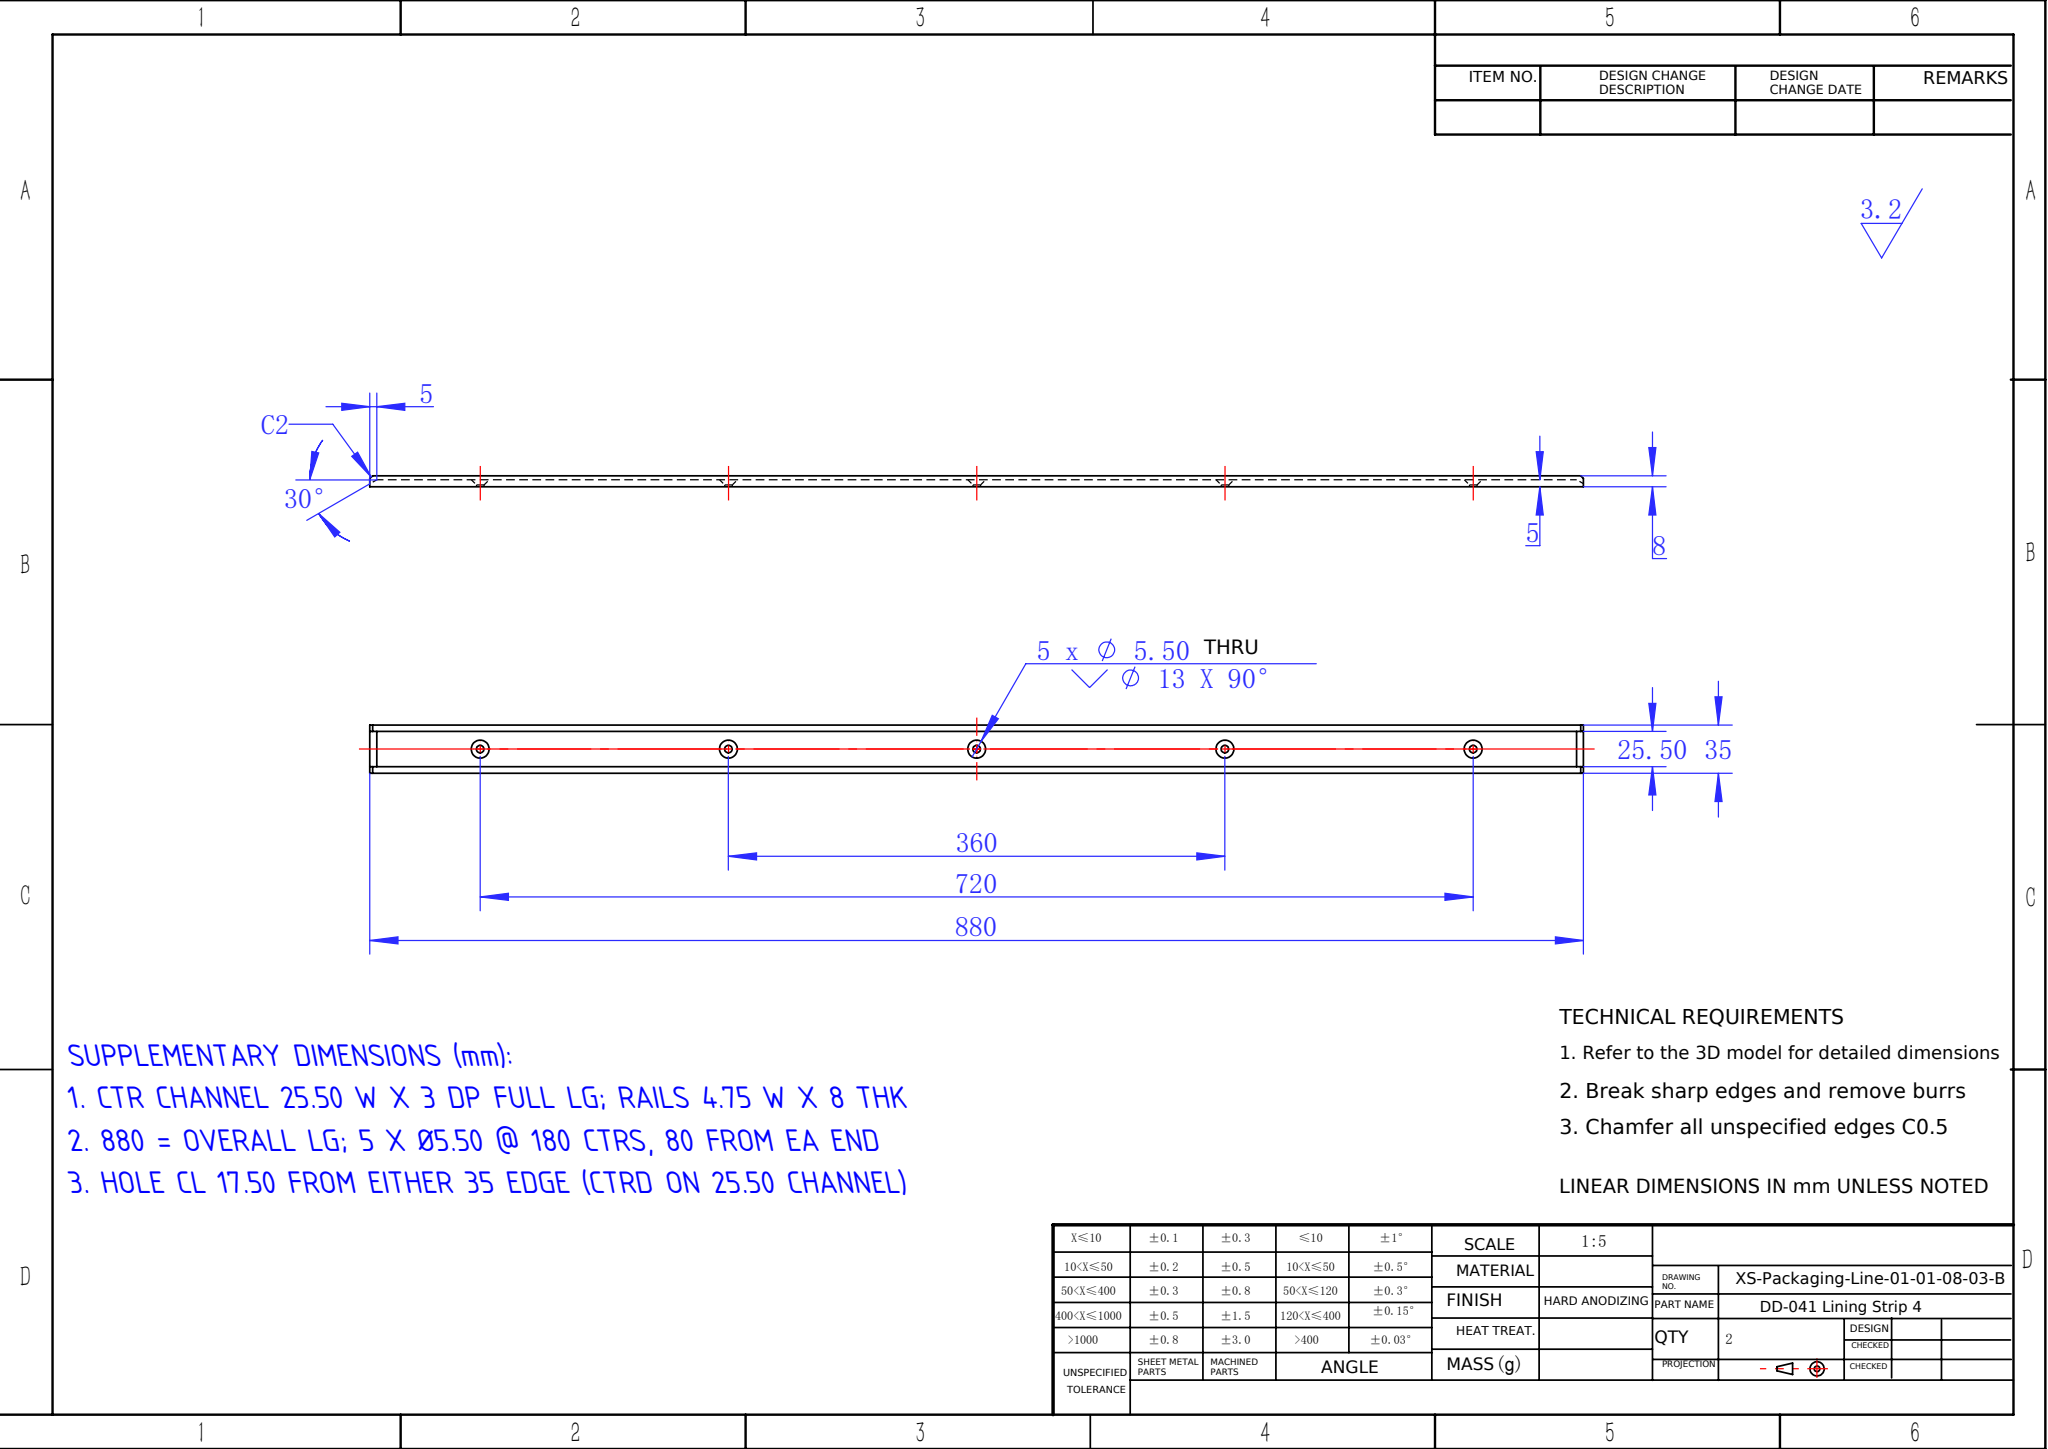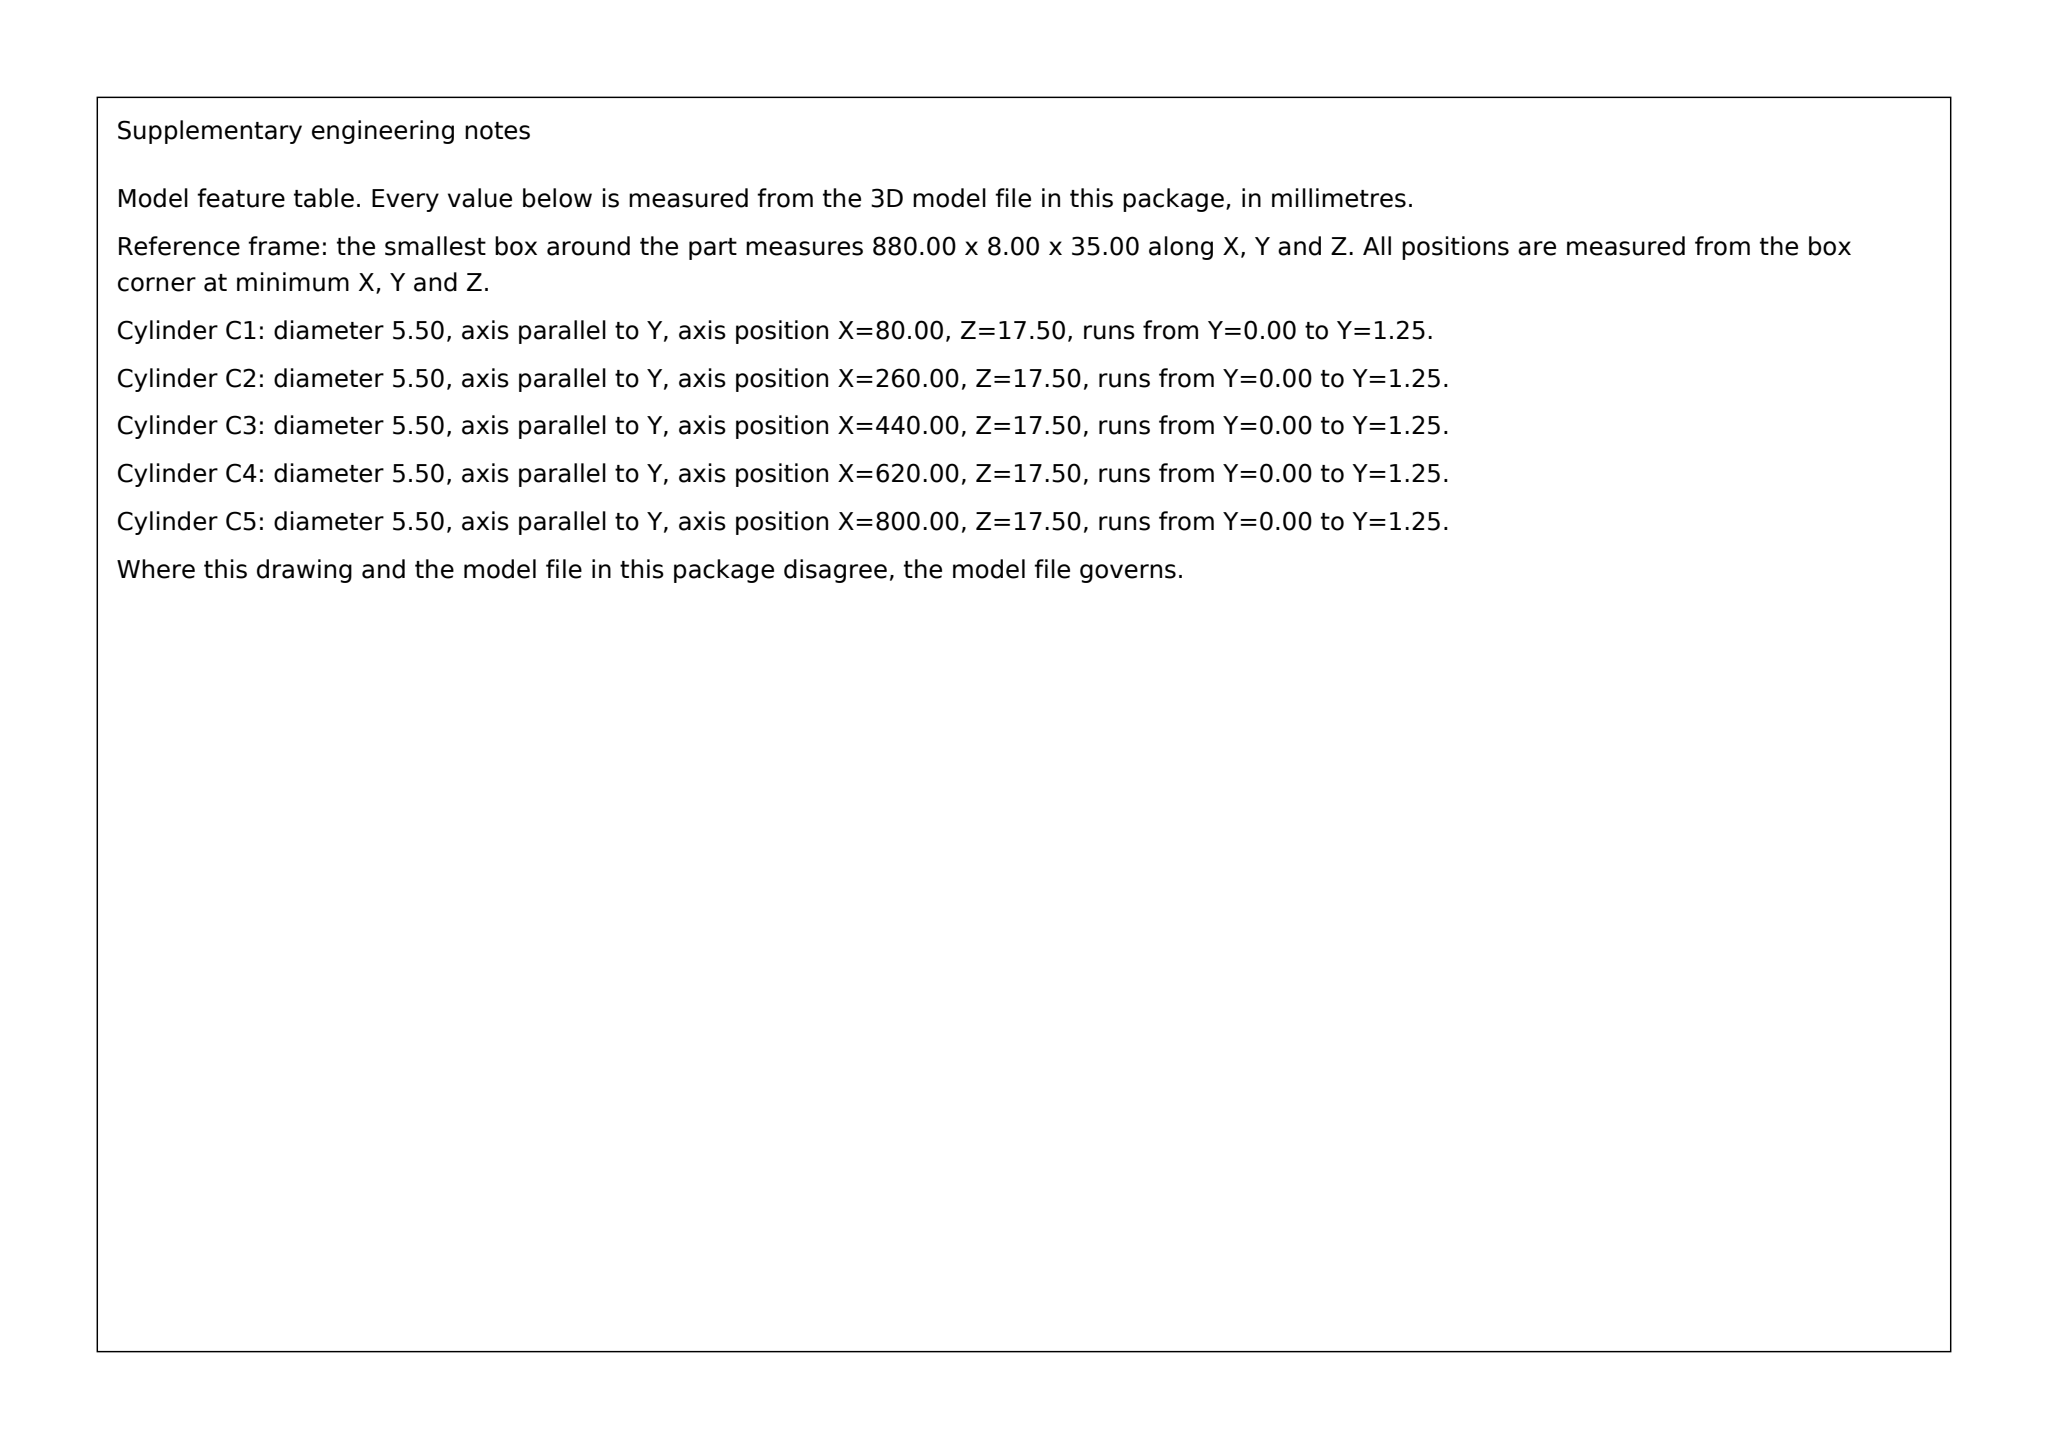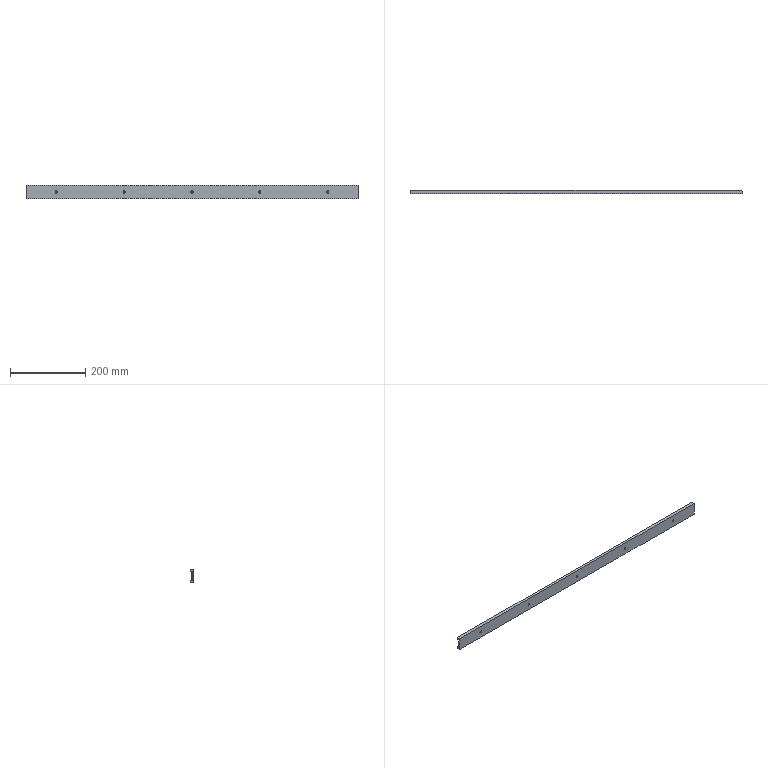Part | SolidWorks | mm | 1 solid | 36 faces | box 880 x 8 x 35 mm | volume 177196 mm3 | plane 16 | cone 10 | cylinder 10 | commonest cylinder face diameters 5.5 x10
build123d program:
from build123d import *

# Parameters (mm, degrees)
SKETCH1_W                                    = 35
SKETCH1_H                                    = 8
BOSS_EXTRUDE1_DEPTH                          = 880
SKETCH2_W                                    = 25.5
SKETCH2_H                                    = 3
CUT_EXTRUDE1_DEPTH                           = 881.732
CHAMFER1_SIZE                                = 5
CHAMFER1_SIZE2                               = 2.887
CHAMFER2_SIZE                                = 5
CHAMFER2_SIZE2                               = 2.887
CHAMFER3_SIZE                                = 2
COUNTERSUNK_HOLE_FOR_M5_HEXAGON_SOCK_2_COUNT = 2
COUNTERSUNK_HOLE_FOR_M5_HEXAGON_SOCK_2_PITCH = 180
COUNTERSUNK_HOLE_FOR_M5_HEXAGON_SOCK_3_COUNT = 2
COUNTERSUNK_HOLE_FOR_M5_HEXAGON_SOCK_3_PITCH = 180
COUNTERSUNK_HOLE_FOR_M5_HEXAGON_SOCK_4_COUNT = 2
COUNTERSUNK_HOLE_FOR_M5_HEXAGON_SOCK_4_PITCH = 360
COUNTERSUNK_HOLE_FOR_M5_HEXAGON_SOCK_5_COUNT = 2
COUNTERSUNK_HOLE_FOR_M5_HEXAGON_SOCK_5_PITCH = 360


with BuildPart() as part:
    # Sketch1 → Boss-Extrude1 (new body)
    with BuildSketch(Plane(origin=(0, 0, 0), x_dir=(0, 0, -1), z_dir=(1, 0, 0))):
        with Locations((17.5, 4)):
            Rectangle(SKETCH1_W, SKETCH1_H)
    extrude(amount=BOSS_EXTRUDE1_DEPTH)

    # Sketch2 → Cut-Extrude1 (cut, through all)
    with BuildSketch(Plane.ZY):
        with Locations((-17.5, 6.5)):
            Rectangle(SKETCH2_W, SKETCH2_H)
    extrude(amount=-CUT_EXTRUDE1_DEPTH, mode=Mode.SUBTRACT)

    # Chamfer1
    chamfer1_edges = [part.edges().sort_by_distance(p)[0] for p in [
        (0, 5, -17.5),
    ]]
    chamfer1_side = [part.faces().sort_by_distance(p)[0] for p in [
        (440, 5, -17.5),
    ]]
    chamfer(chamfer1_edges, length=CHAMFER1_SIZE, length2=CHAMFER1_SIZE2, reference=chamfer1_side[0])

    # Chamfer2
    chamfer2_edges = [part.edges().sort_by_distance(p)[0] for p in [
        (880, 5, -17.5),
    ]]
    chamfer2_side = [part.faces().sort_by_distance(p)[0] for p in [
        (442.5, 5, -17.5),
    ]]
    chamfer(chamfer2_edges, length=CHAMFER2_SIZE, length2=CHAMFER2_SIZE2, reference=chamfer2_side[0])

    # Chamfer3
    chamfer3_edges = [part.edges().sort_by_distance(p)[0] for p in [
        (0, 8, -2.375),
        (880, 8, -2.375),
        (880, 8, -32.625),
        (0, 8, -32.625),
    ]]
    chamfer(chamfer3_edges, length=CHAMFER3_SIZE)

    # Sketch3 → Countersunk Hole for M5 Hexagon Socket C (revolve, cut)
    with BuildSketch(Plane(origin=(440, 5, -17.5), x_dir=(0, 0, 1), z_dir=(1, 0, 0))):
        Polygon((0, 0), (0, 5), (2.75, 5), (2.75, 3.75), (6.5, 0), align=None)
    countersunk_hole_for_m5_hexagon_socket_c = revolve(axis=Axis((440, 11.35, -17.5), (0, -1, 0)), mode=Mode.SUBTRACT)

    # Countersunk Hole for M5 Hexagon Sock 2: Countersunk Hole for M5 Hexagon Socket C ×2
    with Locations(*[(-i * COUNTERSUNK_HOLE_FOR_M5_HEXAGON_SOCK_2_PITCH, 0, 0) for i in range(1, COUNTERSUNK_HOLE_FOR_M5_HEXAGON_SOCK_2_COUNT)]):
        add(countersunk_hole_for_m5_hexagon_socket_c, mode=Mode.SUBTRACT)

    # Countersunk Hole for M5 Hexagon Sock 3: Countersunk Hole for M5 Hexagon Socket C ×2
    with Locations(*[(i * COUNTERSUNK_HOLE_FOR_M5_HEXAGON_SOCK_3_PITCH, 0, 0) for i in range(1, COUNTERSUNK_HOLE_FOR_M5_HEXAGON_SOCK_3_COUNT)]):
        add(countersunk_hole_for_m5_hexagon_socket_c, mode=Mode.SUBTRACT)

    # Countersunk Hole for M5 Hexagon Sock 4: Countersunk Hole for M5 Hexagon Socket C ×2
    with Locations(*[(-i * COUNTERSUNK_HOLE_FOR_M5_HEXAGON_SOCK_4_PITCH, 0, 0) for i in range(1, COUNTERSUNK_HOLE_FOR_M5_HEXAGON_SOCK_4_COUNT)]):
        add(countersunk_hole_for_m5_hexagon_socket_c, mode=Mode.SUBTRACT)

    # Countersunk Hole for M5 Hexagon Sock 5: Countersunk Hole for M5 Hexagon Socket C ×2
    with Locations(*[(i * COUNTERSUNK_HOLE_FOR_M5_HEXAGON_SOCK_5_PITCH, 0, 0) for i in range(1, COUNTERSUNK_HOLE_FOR_M5_HEXAGON_SOCK_5_COUNT)]):
        add(countersunk_hole_for_m5_hexagon_socket_c, mode=Mode.SUBTRACT)


with BuildPart() as part_1:
    # Body-Move_Copy1: moved
    add(part.part.moved(Location((-31.487, 4.557, 0))))


solid = part_1.part